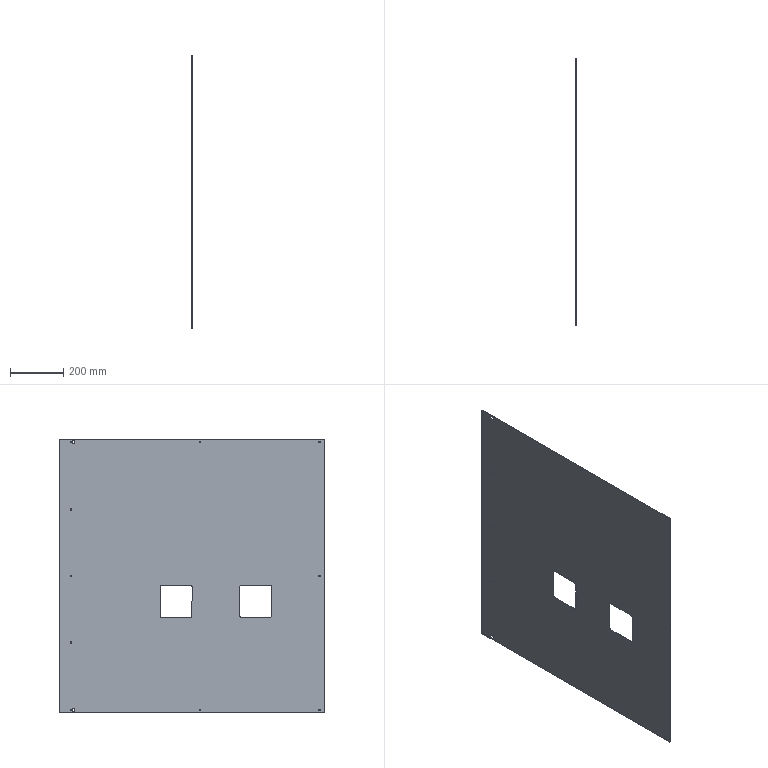Component | SolidWorks | SYM0671-81-104-2 | 1 solid | 50 faces | box 1.2 x 1000 x 1030 mm | volume 1200875 mm3 | cylinder 32 | plane 18 | commonest cylinder face diameters 6 x18 10 x8 12 x6
build123d program:
from build123d import *

# Parameters (mm, degrees)
SKETCH1_2_W               = 1030
SKETCH1_2_H               = 1000
EXTRUDE1_DEPTH            = 1.2
SKETCH2_R                 = 3
EXTRUDE2_DEPTH            = 718.793
LPATTERN1_COUNT           = 2
LPATTERN1_PITCH           = 1010
LPATTERN2_COUNT           = 2
LPATTERN2_PITCH           = 450
LPATTERN2_COPY_1_SKETCH_R = 3
LPATTERN2_COPY_1_DEPTH    = 718.793
SKETCH3_R                 = 3
EXTRUDE3_DEPTH            = 718.793
LPATTERN3_COUNT           = 2
LPATTERN3_PITCH           = 935
EXTRUDE4_DEPTH            = 718.793
LPATTERN4_COUNT           = 2
LPATTERN4_PITCH           = 1010
SKETCH6_W                 = 120
SKETCH6_H                 = 120
EXTRUDE5_DEPTH            = 718.793
FILLET1_R                 = 5
SKETCH1_R                 = 3
CUT_EXTRUDE1_DEPTH        = 718.793


with BuildPart() as part:
    # Sketch1_2 → Extrude1 (new body)
    with BuildSketch(Plane.XY):
        Rectangle(SKETCH1_2_W, SKETCH1_2_H)
    extrude(amount=EXTRUDE1_DEPTH)

    # Sketch2 → Extrude2 (cut, through all)
    with BuildSketch(Plane.XY.offset(1.2)):
        with Locations((-505, -480)):
            Circle(SKETCH2_R)
    extrude2 = extrude(amount=-EXTRUDE2_DEPTH, mode=Mode.SUBTRACT)

    # LPattern1: Extrude2 ×2
    with Locations(*[(i * LPATTERN1_PITCH, 0, 0) for i in range(1, LPATTERN1_COUNT)]):
        add(extrude2, mode=Mode.SUBTRACT)

    # LPattern2: Extrude2 ×2
    with Locations(*[(0, i * LPATTERN2_PITCH, 0) for i in range(1, LPATTERN2_COUNT)]):
        add(extrude2, mode=Mode.SUBTRACT)

    # LPattern2 copy 1 sketch → LPattern2 copy 1 (cut, through all)
    with BuildSketch(Plane(origin=(1010, 450, 1.2), x_dir=(1, 0, 0), z_dir=(0, 0, 1))):
        with Locations((-505, -480)):
            Circle(LPATTERN2_COPY_1_SKETCH_R)
    extrude(amount=-LPATTERN2_COPY_1_DEPTH, mode=Mode.SUBTRACT)

    # Sketch3 → Extrude3 (cut, through all)
    with BuildSketch(Plane.XY.offset(1.2)):
        with Locations((0, -480)):
            Circle(SKETCH3_R)
    extrude3 = extrude(amount=-EXTRUDE3_DEPTH, mode=Mode.SUBTRACT)

    # LPattern3: Extrude3 ×2
    with Locations(*[(0, i * LPATTERN3_PITCH, 0) for i in range(1, LPATTERN3_COUNT)]):
        add(extrude3, mode=Mode.SUBTRACT)

    # Sketch4 → Extrude4 (cut, through all)
    with BuildSketch(Plane.XY.offset(1.2)):
        with BuildLine():
            Line((-508, 455), (-508, 451.696))
            ThreePointArc((-508, 451.696), (-505, 440.5), (-502, 451.696))
            Line((-502, 451.696), (-502, 455))
            ThreePointArc((-502, 455), (-505, 458), (-508, 455))
        make_face()
    extrude4 = extrude(amount=-EXTRUDE4_DEPTH, mode=Mode.SUBTRACT)

    # LPattern4: Extrude4 ×2
    with Locations(*[(i * LPATTERN4_PITCH, 0, 0) for i in range(1, LPATTERN4_COUNT)]):
        add(extrude4, mode=Mode.SUBTRACT)

    # Sketch6 → Extrude5 (cut, through all)
    with BuildSketch(Plane.XY.offset(1.2)):
        with Locations((-95, -240)):
            Rectangle(SKETCH6_W, SKETCH6_H)
        with Locations((-95, 60)):
            Rectangle(SKETCH6_W, SKETCH6_H)
    extrude(amount=-EXTRUDE5_DEPTH, mode=Mode.SUBTRACT)

    # Fillet1
    fillet1_edges = [part.edges().sort_by_distance(p)[0] for p in [
        (-155, -300, 0.6),
        (-155, -180, 0.6),
        (-35, -180, 0.6),
        (-35, -300, 0.6),
        (-155, 0, 0.6),
        (-155, 120, 0.6),
        (-35, 120, 0.6),
        (-35, 0, 0.6),
    ]]
    fillet(fillet1_edges, radius=FILLET1_R)

    # Sketch1 → Cut-Extrude1 (cut, through all)
    with BuildSketch(Plane.XY.offset(1.2)):
        with Locations((-250, 455)):
            Circle(SKETCH1_R)
        with Locations((250, 455)):
            Circle(SKETCH1_R)
    extrude(amount=-CUT_EXTRUDE1_DEPTH, mode=Mode.SUBTRACT)


solid = part.part

# Placed as in the assembly
solid = solid.moved(Location((548.451, -16.857, 515.518), (0, -90, 0)))